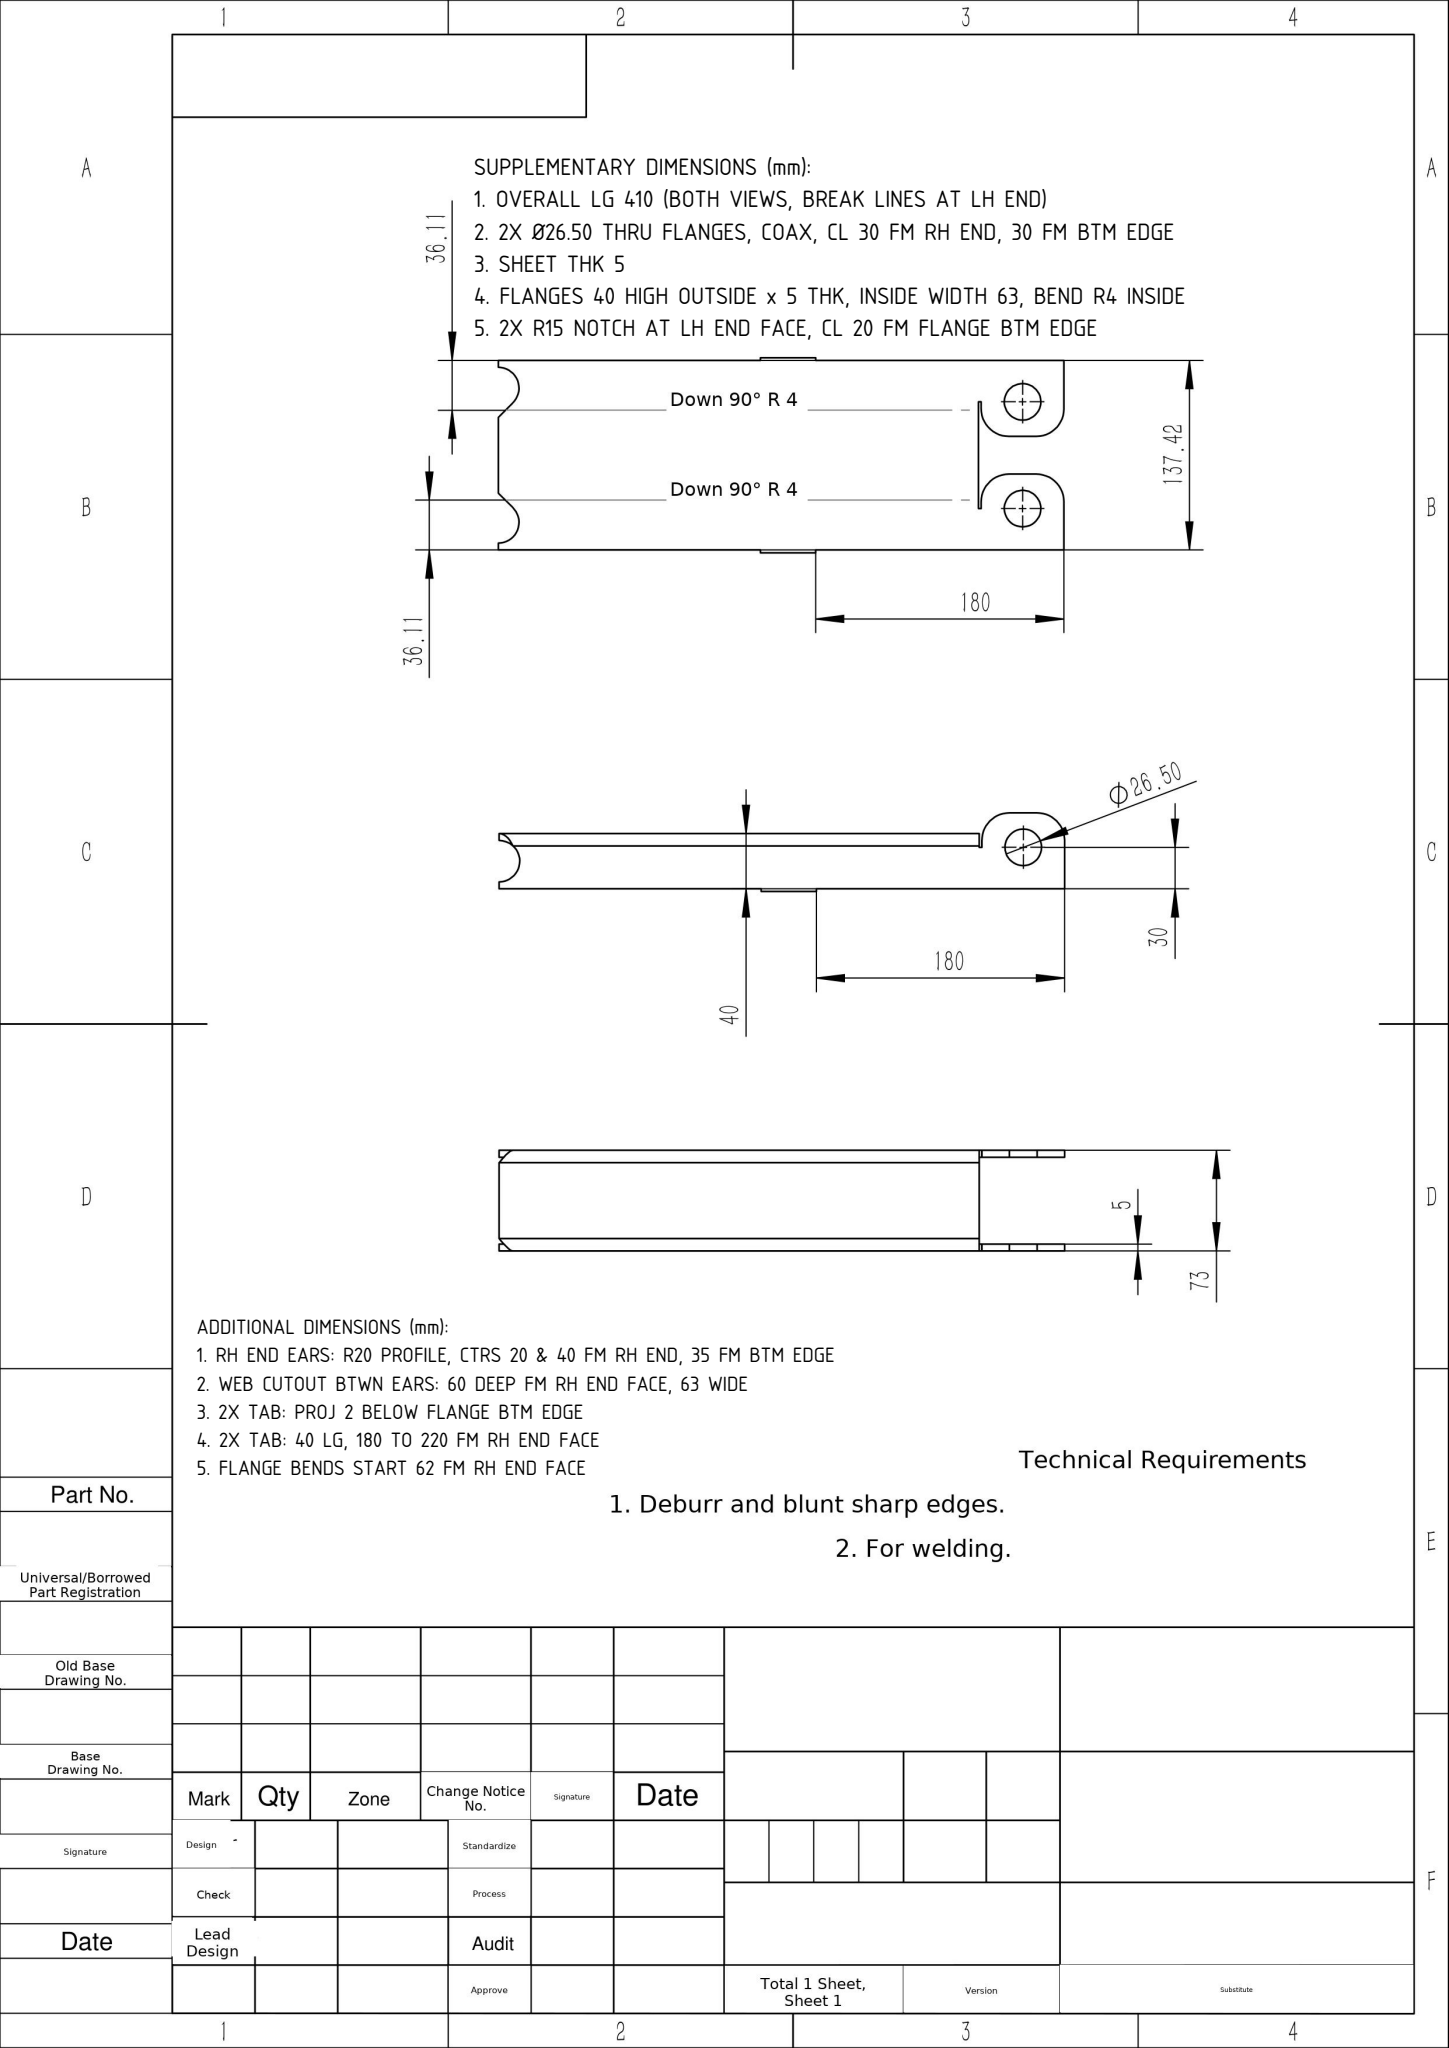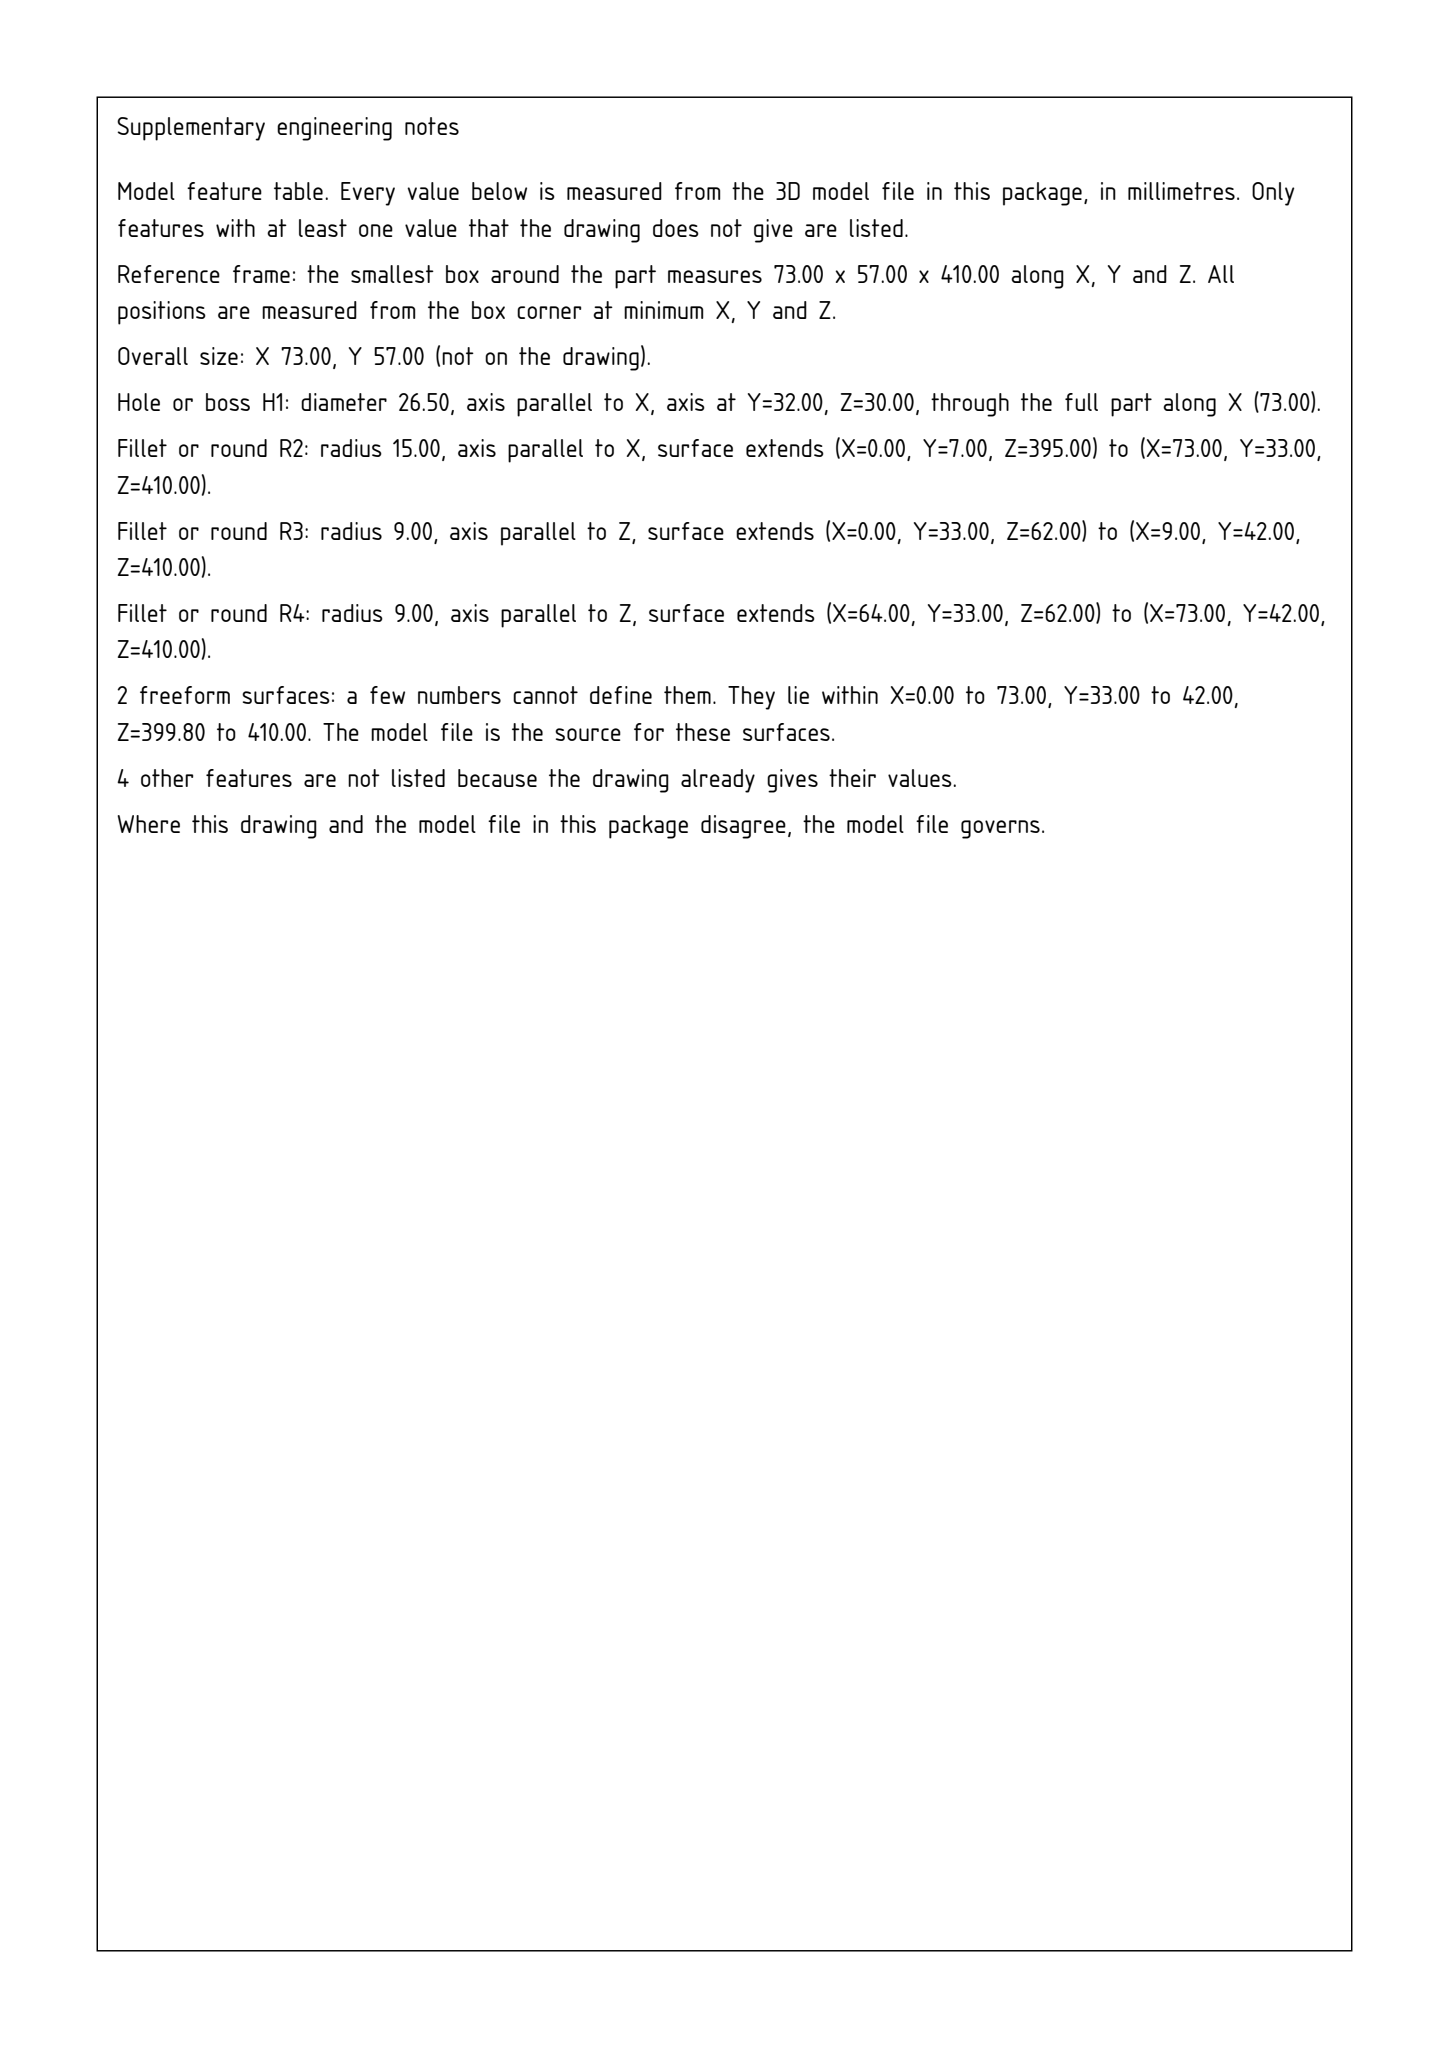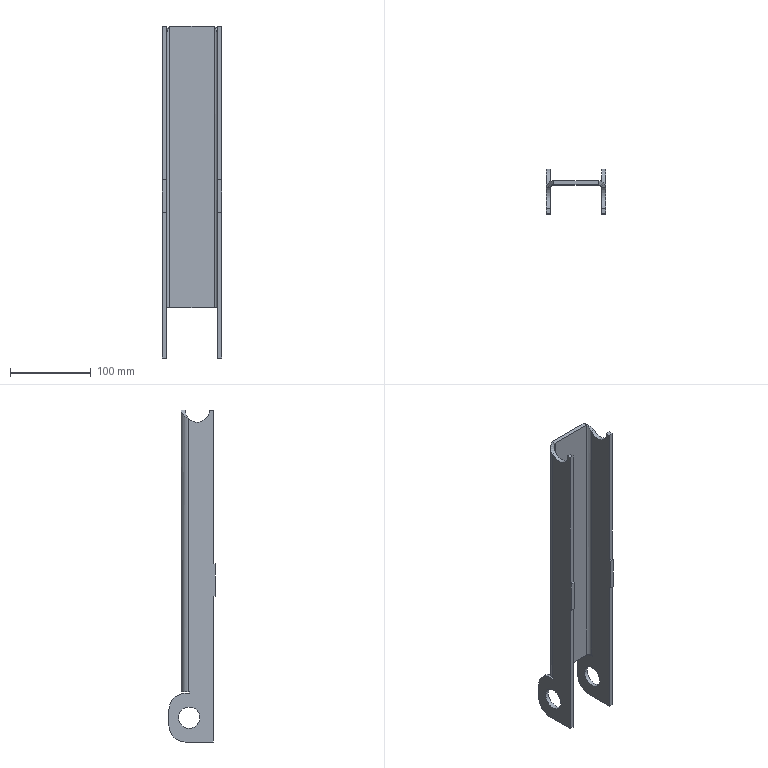Part | SolidWorks | mm | 1 solid | 44 faces | box 73 x 57 x 410 mm | volume 262456 mm3 | plane 28 | cylinder 14 | spline 2 | commonest cylinder face diameters 26.5 x4 40 x4 8 x2 18 x2 30 x2